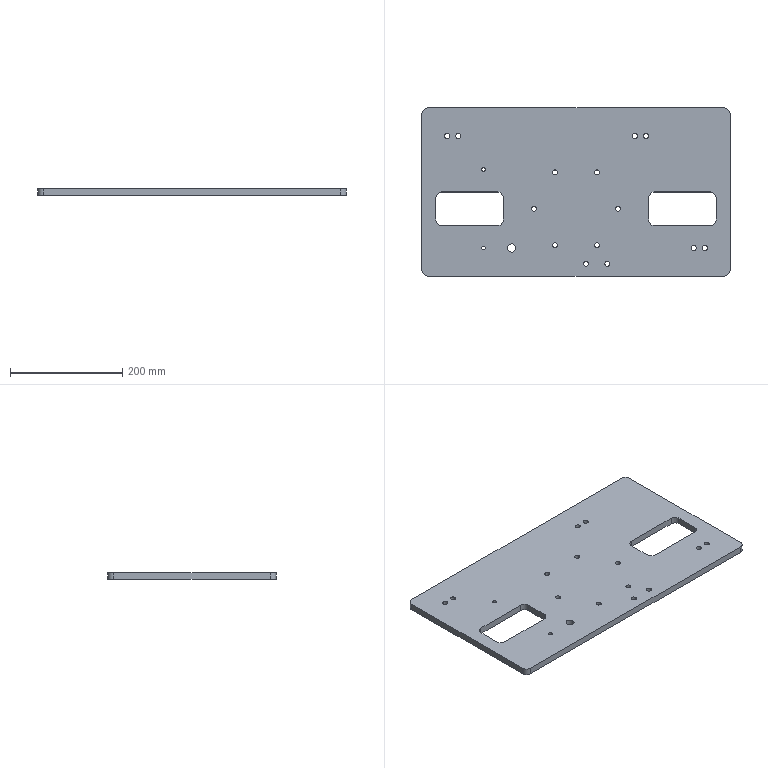Component | SolidWorks | CylinderBasePlate2-1 | 1 solid | 72 faces | box 550 x 300 x 12 mm | volume 1748398 mm3 | cylinder 52 | plane 20 | commonest cylinder face diameters 9 x28 20 x12 6.8 x4 4 x4 14.5 x2 170 x2 | material 6063
build123d program:
from build123d import *

# Parameters (mm, degrees)
SKETCH1_W                  = 550
SKETCH1_H                  = 300
BOSS_EXTRUDE1_DEPTH        = 12
SKETCH6_R                  = 85
CUT_EXTRUDE3_DEPTH         = 2
SKETCH7_R                  = 4.5
CUT_EXTRUDE4_DEPTH         = 314.409
FILLET1_R                  = 10
M8_TAPPED_HOLE1_D          = 6.8
M8_TAPPED_HOLE1_DEPTH      = 19.75
M8_TAPPED_HOLE1_TIP        = 2.043
SKETCH9_W                  = 120
SKETCH9_H                  = 60
CUT_EXTRUDE7_DEPTH         = 314.479
FILLET2_R                  = 10
SKETCH11_R                 = 4.5
CUT_EXTRUDE8_DEPTH         = 314.479
M16X1_5_TAPPED_HOLE1_D     = 14.5
M16X1_5_TAPPED_HOLE1_DEPTH = 36.5
M16X1_5_TAPPED_HOLE1_TIP   = 4.356
SKETCH14_W                 = 80
SKETCH14_H                 = 12
CUT_EXTRUDE9_DEPTH         = 2
SKETCH15_R                 = 4.5
CUT_EXTRUDE10_DEPTH        = 314.409
FILLET3_R                  = 2


with BuildPart() as part:
    # Sketch1 → Boss-Extrude1 (new body)
    with BuildSketch(Plane.XY):
        Rectangle(SKETCH1_W, SKETCH1_H)
    extrude(amount=BOSS_EXTRUDE1_DEPTH)

    # Sketch6 → Cut-Extrude3 (cut)
    with BuildSketch(Plane(origin=(0, 0, 0), x_dir=(-1, 0, 0), z_dir=(0, 0, -1))):
        with Locations((0, -30)):
            Circle(SKETCH6_R)
    extrude(amount=-CUT_EXTRUDE3_DEPTH, mode=Mode.SUBTRACT)

    # Sketch7 → Cut-Extrude4 (cut, through all)
    with BuildSketch(Plane(origin=(0, 0, 2), x_dir=(-1, 0, 0), z_dir=(0, 0, -1))):
        with Locations((-37.5, 34.952)):
            Circle(SKETCH7_R)
        with Locations((37.5, 34.952)):
            Circle(SKETCH7_R)
        with Locations((75, -30)):
            Circle(SKETCH7_R)
        with Locations((-75, -30)):
            Circle(SKETCH7_R)
        with Locations((-37.5, -94.952)):
            Circle(SKETCH7_R)
        with Locations((37.5, -94.952)):
            Circle(SKETCH7_R)
    extrude(amount=-CUT_EXTRUDE4_DEPTH, mode=Mode.SUBTRACT)

    # Fillet1
    fillet1_edges = [part.edges().sort_by_distance(p)[0] for p in [
        (275, -150, 6),
        (-275, -150, 6),
        (-275, 150, 6),
        (275, 150, 6),
    ]]
    fillet(fillet1_edges, radius=FILLET1_R)

    # M8 Tapped Hole1
    with Locations(Plane(origin=(-165, 40, 12), x_dir=(1, 0, 0), z_dir=(0, 0, 1))):
        with Locations((0, 0), (0, -140)):
            Hole(M8_TAPPED_HOLE1_D / 2, depth=M8_TAPPED_HOLE1_DEPTH)
            with Locations((0, 0, -(M8_TAPPED_HOLE1_DEPTH + M8_TAPPED_HOLE1_TIP / 2))):  # 118° drill point
                Cone(0, M8_TAPPED_HOLE1_D / 2, M8_TAPPED_HOLE1_TIP, mode=Mode.SUBTRACT)

    # Sketch9 → Cut-Extrude7 (cut, through all)
    with BuildSketch(Plane.XY.offset(12)):
        with Locations((-190, -30)):
            Rectangle(SKETCH9_W, SKETCH9_H)
        with Locations((190, -30)):
            Rectangle(SKETCH9_W, SKETCH9_H)
    extrude(amount=-CUT_EXTRUDE7_DEPTH, mode=Mode.SUBTRACT)

    # Fillet2
    fillet2_edges = [part.edges().sort_by_distance(p)[0] for p in [
        (-130, 0, 6),
        (-130, -60, 6),
        (-250, -60, 6),
        (-250, 0, 6),
        (250, 0, 6),
        (250, -60, 6),
        (130, -60, 6),
        (130, 0, 6),
    ]]
    fillet(fillet2_edges, radius=FILLET2_R)

    # Sketch11 → Cut-Extrude8 (cut, through all)
    with BuildSketch(Plane.XY.offset(12)):
        with Locations((210, -100)):
            Circle(SKETCH11_R)
        with Locations((230, -100)):
            Circle(SKETCH11_R)
        with Locations((125, 100)):
            Circle(SKETCH11_R)
        with Locations((105, 100)):
            Circle(SKETCH11_R)
        with Locations((-230, 100)):
            Circle(SKETCH11_R)
        with Locations((-210, 100)):
            Circle(SKETCH11_R)
    extrude(amount=-CUT_EXTRUDE8_DEPTH, mode=Mode.SUBTRACT)

    # M16x1.5 Tapped Hole1
    with Locations(Plane(origin=(-115, -100, 12), x_dir=(1, 0, 0), z_dir=(0, 0, 1))):
        with Locations((0, 0)):
            Hole(M16X1_5_TAPPED_HOLE1_D / 2, depth=M16X1_5_TAPPED_HOLE1_DEPTH)
            with Locations((0, 0, -(M16X1_5_TAPPED_HOLE1_DEPTH + M16X1_5_TAPPED_HOLE1_TIP / 2))):  # 118° drill point
                Cone(0, M16X1_5_TAPPED_HOLE1_D / 2, M16X1_5_TAPPED_HOLE1_TIP, mode=Mode.SUBTRACT)

    # Sketch14 → Cut-Extrude9 (cut)
    with BuildSketch(Plane(origin=(0, 0, 0), x_dir=(-1, 0, 0), z_dir=(0, 0, -1))):
        with Locations((-37, -128)):
            Rectangle(SKETCH14_W, SKETCH14_H)
    extrude(amount=-CUT_EXTRUDE9_DEPTH, mode=Mode.SUBTRACT)

    # Sketch15 → Cut-Extrude10 (cut, through all)
    with BuildSketch(Plane(origin=(0, 0, 2), x_dir=(-1, 0, 0), z_dir=(0, 0, -1))):
        with Locations((-56, -128)):
            Circle(SKETCH15_R)
        with Locations((-18, -128)):
            Circle(SKETCH15_R)
    extrude(amount=-CUT_EXTRUDE10_DEPTH, mode=Mode.SUBTRACT)

    # Fillet3
    fillet3_edges = [part.edges().sort_by_distance(p)[0] for p in [
        (-3, -122, 1),
        (-3, -134, 1),
        (77, -134, 1),
        (77, -122, 1),
    ]]
    fillet(fillet3_edges, radius=FILLET3_R)


solid = part.part

# Placed as in the assembly
solid = solid.moved(Location((1.785, 3.083, -1192.957), (0, 0, 0)))